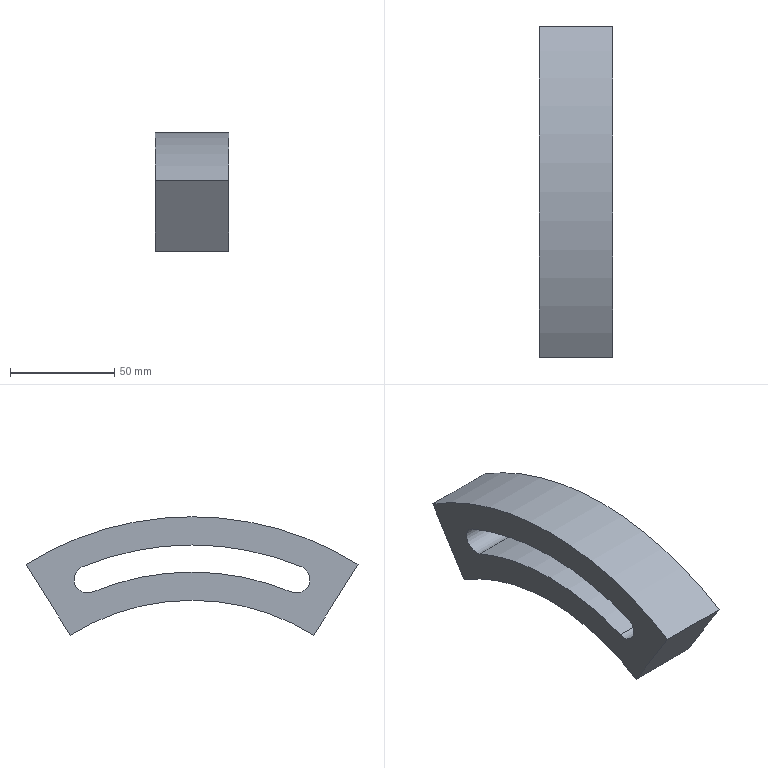Component | NX | COUNTERWEIGHT_BLOCK | 1 solid | 10 faces | box 35 x 158.98 x 56.71 mm | volume 151947 mm3 | cylinder 6 | plane 4 | commonest cylinder face diameters 13 x2 220 x1 300 x1 273 x1 247 x1
STEP:
#1=CARTESIAN_POINT('',(0.,0.,0.));
#2=DIRECTION('',(0.,0.,1.));
#3=DIRECTION('',(1.,0.,0.));
#4=AXIS2_PLACEMENT_3D('',#1,#2,#3);
#5=CARTESIAN_POINT('',(505.625,-79.397,126.65));
#6=VERTEX_POINT('',#5);
#7=CARTESIAN_POINT('',(505.625,-58.2,92.728));
#8=VERTEX_POINT('',#7);
#9=CARTESIAN_POINT('',(505.625,-79.397,126.65));
#10=DIRECTION('',(0.,0.5299,-0.848));
#11=VECTOR('',#10,1.);
#12=LINE('',#9,#11);
#13=CARTESIAN_POINT('',(540.625,-79.397,126.65));
#14=DIRECTION('',(0.,0.848,0.5299));
#15=DIRECTION('',(0.,-0.5299,0.848));
#16=AXIS2_PLACEMENT_3D('',#13,#14,#15);
#17=PLANE('',#16);
#18=CARTESIAN_POINT('',(0.,-35.));
#19=DIRECTION('',(-1.,0.));
#20=VECTOR('',#19,1.);
#21=LINE('',#18,#20);
#22=(GEOMETRIC_REPRESENTATION_CONTEXT(2)PARAMETRIC_REPRESENTATION_CONTEXT()REPRESENTATION_CONTEXT('',''));
#23=DEFINITIONAL_REPRESENTATION('',(#21),#22);
#24=PCURVE('',#17,#23);
#25=CARTESIAN_POINT('',(505.625,0.09065,-0.557));
#26=DIRECTION('',(-1.,0.,0.));
#27=DIRECTION('',(0.,0.,1.));
#28=AXIS2_PLACEMENT_3D('',#25,#26,#27);
#29=PLANE('',#28);
#30=CARTESIAN_POINT('',(127.207,-79.488));
#31=DIRECTION('',(-0.848,0.5299));
#32=VECTOR('',#31,1.);
#33=LINE('',#30,#32);
#34=(GEOMETRIC_REPRESENTATION_CONTEXT(2)PARAMETRIC_REPRESENTATION_CONTEXT()REPRESENTATION_CONTEXT('',''));
#35=DEFINITIONAL_REPRESENTATION('',(#33),#34);
#36=PCURVE('',#29,#35);
#37=SURFACE_CURVE('',#12,(#24,#36),.PCURVE_S1.);
#38=EDGE_CURVE('',#6,#8,#37,.T.);
#39=ORIENTED_EDGE('',*,*,#38,.T.);
#40=CARTESIAN_POINT('',(540.625,-58.2,92.728));
#41=VERTEX_POINT('',#40);
#42=CARTESIAN_POINT('',(540.625,-58.2,92.728));
#43=DIRECTION('',(-1.,0.,0.));
#44=VECTOR('',#43,1.);
#45=LINE('',#42,#44);
#46=CARTESIAN_POINT('',(-40.,0.));
#47=DIRECTION('',(0.,-1.));
#48=VECTOR('',#47,1.);
#49=LINE('',#46,#48);
#50=(GEOMETRIC_REPRESENTATION_CONTEXT(2)PARAMETRIC_REPRESENTATION_CONTEXT()REPRESENTATION_CONTEXT('',''));
#51=DEFINITIONAL_REPRESENTATION('',(#49),#50);
#52=PCURVE('',#17,#51);
#53=CARTESIAN_POINT('',(540.625,0.09065,-0.557));
#54=DIRECTION('',(-1.,0.,0.));
#55=DIRECTION('',(0.,0.,1.));
#56=AXIS2_PLACEMENT_3D('',#53,#54,#55);
#57=CYLINDRICAL_SURFACE('',#56,110.);
#58=CARTESIAN_POINT('',(-0.5585,0.));
#59=DIRECTION('',(0.,1.));
#60=VECTOR('',#59,1.);
#61=LINE('',#58,#60);
#62=(GEOMETRIC_REPRESENTATION_CONTEXT(2)PARAMETRIC_REPRESENTATION_CONTEXT()REPRESENTATION_CONTEXT('',''));
#63=DEFINITIONAL_REPRESENTATION('',(#61),#62);
#64=PCURVE('',#57,#63);
#65=SURFACE_CURVE('',#45,(#52,#64),.PCURVE_S1.);
#66=EDGE_CURVE('',#41,#8,#65,.T.);
#67=ORIENTED_EDGE('',*,*,#66,.F.);
#68=CARTESIAN_POINT('',(540.625,-79.397,126.65));
#69=VERTEX_POINT('',#68);
#70=CARTESIAN_POINT('',(540.625,-79.397,126.65));
#71=DIRECTION('',(0.,0.5299,-0.848));
#72=VECTOR('',#71,1.);
#73=LINE('',#70,#72);
#74=CARTESIAN_POINT('',(0.,0.));
#75=DIRECTION('',(-1.,0.));
#76=VECTOR('',#75,1.);
#77=LINE('',#74,#76);
#78=(GEOMETRIC_REPRESENTATION_CONTEXT(2)PARAMETRIC_REPRESENTATION_CONTEXT()REPRESENTATION_CONTEXT('',''));
#79=DEFINITIONAL_REPRESENTATION('',(#77),#78);
#80=PCURVE('',#17,#79);
#81=CARTESIAN_POINT('',(540.625,0.09065,-0.557));
#82=DIRECTION('',(-1.,0.,0.));
#83=DIRECTION('',(0.,0.,1.));
#84=AXIS2_PLACEMENT_3D('',#81,#82,#83);
#85=PLANE('',#84);
#86=CARTESIAN_POINT('',(127.207,-79.488));
#87=DIRECTION('',(-0.848,0.5299));
#88=VECTOR('',#87,1.);
#89=LINE('',#86,#88);
#90=(GEOMETRIC_REPRESENTATION_CONTEXT(2)PARAMETRIC_REPRESENTATION_CONTEXT()REPRESENTATION_CONTEXT('',''));
#91=DEFINITIONAL_REPRESENTATION('',(#89),#90);
#92=PCURVE('',#85,#91);
#93=SURFACE_CURVE('',#73,(#80,#92),.PCURVE_S1.);
#94=EDGE_CURVE('',#69,#41,#93,.T.);
#95=ORIENTED_EDGE('',*,*,#94,.F.);
#96=CARTESIAN_POINT('',(540.625,-79.397,126.65));
#97=DIRECTION('',(-1.,0.,0.));
#98=VECTOR('',#97,1.);
#99=LINE('',#96,#98);
#100=CARTESIAN_POINT('',(0.,0.));
#101=DIRECTION('',(0.,-1.));
#102=VECTOR('',#101,1.);
#103=LINE('',#100,#102);
#104=(GEOMETRIC_REPRESENTATION_CONTEXT(2)PARAMETRIC_REPRESENTATION_CONTEXT()REPRESENTATION_CONTEXT('',''));
#105=DEFINITIONAL_REPRESENTATION('',(#103),#104);
#106=PCURVE('',#17,#105);
#107=CARTESIAN_POINT('',(540.625,0.09065,-0.557));
#108=DIRECTION('',(-1.,0.,0.));
#109=DIRECTION('',(0.,0.,1.));
#110=AXIS2_PLACEMENT_3D('',#107,#108,#109);
#111=CYLINDRICAL_SURFACE('',#110,150.);
#112=CARTESIAN_POINT('',(-0.5585,0.));
#113=DIRECTION('',(0.,1.));
#114=VECTOR('',#113,1.);
#115=LINE('',#112,#114);
#116=(GEOMETRIC_REPRESENTATION_CONTEXT(2)PARAMETRIC_REPRESENTATION_CONTEXT()REPRESENTATION_CONTEXT('',''));
#117=DEFINITIONAL_REPRESENTATION('',(#115),#116);
#118=PCURVE('',#111,#117);
#119=SURFACE_CURVE('',#99,(#106,#118),.PCURVE_S1.);
#120=EDGE_CURVE('',#69,#6,#119,.T.);
#121=ORIENTED_EDGE('',*,*,#120,.T.);
#122=EDGE_LOOP('',(#39,#67,#95,#121));
#123=FACE_BOUND('',#122,.T.);
#124=ADVANCED_FACE('',(#123),#17,.F.);
#125=ORIENTED_EDGE('',*,*,#66,.F.);
#126=CARTESIAN_POINT('',(540.625,58.382,92.728));
#127=VERTEX_POINT('',#126);
#128=CARTESIAN_POINT('',(540.625,0.09065,-0.557));
#129=DIRECTION('',(-1.,0.,0.));
#130=DIRECTION('',(0.,1.,0.));
#131=AXIS2_PLACEMENT_3D('',#128,#129,#130);
#132=CIRCLE('',#131,110.);
#133=CARTESIAN_POINT('',(-4.712,0.));
#134=DIRECTION('',(1.,0.));
#135=VECTOR('',#134,1.);
#136=LINE('',#133,#135);
#137=(GEOMETRIC_REPRESENTATION_CONTEXT(2)PARAMETRIC_REPRESENTATION_CONTEXT()REPRESENTATION_CONTEXT('',''));
#138=DEFINITIONAL_REPRESENTATION('',(#136),#137);
#139=PCURVE('',#57,#138);
#140=CARTESIAN_POINT('',(0.,0.));
#141=DIRECTION('',(0.,1.));
#142=AXIS2_PLACEMENT_2D('',#140,#141);
#143=CIRCLE('',#142,110.);
#144=(GEOMETRIC_REPRESENTATION_CONTEXT(2)PARAMETRIC_REPRESENTATION_CONTEXT()REPRESENTATION_CONTEXT('',''));
#145=DEFINITIONAL_REPRESENTATION('',(#143),#144);
#146=PCURVE('',#85,#145);
#147=SURFACE_CURVE('',#132,(#139,#146),.PCURVE_S1.);
#148=EDGE_CURVE('',#41,#127,#147,.T.);
#149=ORIENTED_EDGE('',*,*,#148,.T.);
#150=CARTESIAN_POINT('',(505.625,58.382,92.728));
#151=VERTEX_POINT('',#150);
#152=CARTESIAN_POINT('',(540.625,58.382,92.728));
#153=DIRECTION('',(-1.,0.,0.));
#154=VECTOR('',#153,1.);
#155=LINE('',#152,#154);
#156=CARTESIAN_POINT('',(0.5585,0.));
#157=DIRECTION('',(0.,1.));
#158=VECTOR('',#157,1.);
#159=LINE('',#156,#158);
#160=(GEOMETRIC_REPRESENTATION_CONTEXT(2)PARAMETRIC_REPRESENTATION_CONTEXT()REPRESENTATION_CONTEXT('',''));
#161=DEFINITIONAL_REPRESENTATION('',(#159),#160);
#162=PCURVE('',#57,#161);
#163=CARTESIAN_POINT('',(540.625,58.382,92.728));
#164=DIRECTION('',(0.,-0.848,0.5299));
#165=DIRECTION('',(0.,-0.5299,-0.848));
#166=AXIS2_PLACEMENT_3D('',#163,#164,#165);
#167=PLANE('',#166);
#168=CARTESIAN_POINT('',(0.,0.));
#169=DIRECTION('',(0.,-1.));
#170=VECTOR('',#169,1.);
#171=LINE('',#168,#170);
#172=(GEOMETRIC_REPRESENTATION_CONTEXT(2)PARAMETRIC_REPRESENTATION_CONTEXT()REPRESENTATION_CONTEXT('',''));
#173=DEFINITIONAL_REPRESENTATION('',(#171),#172);
#174=PCURVE('',#167,#173);
#175=SURFACE_CURVE('',#155,(#162,#174),.PCURVE_S1.);
#176=EDGE_CURVE('',#127,#151,#175,.T.);
#177=ORIENTED_EDGE('',*,*,#176,.T.);
#178=CARTESIAN_POINT('',(505.625,0.09065,-0.557));
#179=DIRECTION('',(-1.,0.,0.));
#180=DIRECTION('',(0.,1.,0.));
#181=AXIS2_PLACEMENT_3D('',#178,#179,#180);
#182=CIRCLE('',#181,110.);
#183=CARTESIAN_POINT('',(-4.712,35.));
#184=DIRECTION('',(1.,0.));
#185=VECTOR('',#184,1.);
#186=LINE('',#183,#185);
#187=(GEOMETRIC_REPRESENTATION_CONTEXT(2)PARAMETRIC_REPRESENTATION_CONTEXT()REPRESENTATION_CONTEXT('',''));
#188=DEFINITIONAL_REPRESENTATION('',(#186),#187);
#189=PCURVE('',#57,#188);
#190=CARTESIAN_POINT('',(0.,0.));
#191=DIRECTION('',(0.,1.));
#192=AXIS2_PLACEMENT_2D('',#190,#191);
#193=CIRCLE('',#192,110.);
#194=(GEOMETRIC_REPRESENTATION_CONTEXT(2)PARAMETRIC_REPRESENTATION_CONTEXT()REPRESENTATION_CONTEXT('',''));
#195=DEFINITIONAL_REPRESENTATION('',(#193),#194);
#196=PCURVE('',#29,#195);
#197=SURFACE_CURVE('',#182,(#189,#196),.PCURVE_S1.);
#198=EDGE_CURVE('',#8,#151,#197,.T.);
#199=ORIENTED_EDGE('',*,*,#198,.F.);
#200=EDGE_LOOP('',(#125,#149,#177,#199));
#201=FACE_BOUND('',#200,.F.);
#202=ADVANCED_FACE('',(#201),#57,.F.);
#203=CARTESIAN_POINT('',(505.625,79.579,126.65));
#204=VERTEX_POINT('',#203);
#205=CARTESIAN_POINT('',(505.625,58.382,92.728));
#206=DIRECTION('',(0.,0.5299,0.848));
#207=VECTOR('',#206,1.);
#208=LINE('',#205,#207);
#209=CARTESIAN_POINT('',(0.,-35.));
#210=DIRECTION('',(-1.,0.));
#211=VECTOR('',#210,1.);
#212=LINE('',#209,#211);
#213=(GEOMETRIC_REPRESENTATION_CONTEXT(2)PARAMETRIC_REPRESENTATION_CONTEXT()REPRESENTATION_CONTEXT('',''));
#214=DEFINITIONAL_REPRESENTATION('',(#212),#213);
#215=PCURVE('',#167,#214);
#216=CARTESIAN_POINT('',(93.285,58.291));
#217=DIRECTION('',(0.848,0.5299));
#218=VECTOR('',#217,1.);
#219=LINE('',#216,#218);
#220=(GEOMETRIC_REPRESENTATION_CONTEXT(2)PARAMETRIC_REPRESENTATION_CONTEXT()REPRESENTATION_CONTEXT('',''));
#221=DEFINITIONAL_REPRESENTATION('',(#219),#220);
#222=PCURVE('',#29,#221);
#223=SURFACE_CURVE('',#208,(#215,#222),.PCURVE_S1.);
#224=EDGE_CURVE('',#151,#204,#223,.T.);
#225=ORIENTED_EDGE('',*,*,#224,.T.);
#226=CARTESIAN_POINT('',(540.625,79.579,126.65));
#227=VERTEX_POINT('',#226);
#228=CARTESIAN_POINT('',(540.625,79.579,126.65));
#229=DIRECTION('',(-1.,0.,0.));
#230=VECTOR('',#229,1.);
#231=LINE('',#228,#230);
#232=CARTESIAN_POINT('',(-40.,0.));
#233=DIRECTION('',(0.,-1.));
#234=VECTOR('',#233,1.);
#235=LINE('',#232,#234);
#236=(GEOMETRIC_REPRESENTATION_CONTEXT(2)PARAMETRIC_REPRESENTATION_CONTEXT()REPRESENTATION_CONTEXT('',''));
#237=DEFINITIONAL_REPRESENTATION('',(#235),#236);
#238=PCURVE('',#167,#237);
#239=CARTESIAN_POINT('',(0.5585,0.));
#240=DIRECTION('',(0.,1.));
#241=VECTOR('',#240,1.);
#242=LINE('',#239,#241);
#243=(GEOMETRIC_REPRESENTATION_CONTEXT(2)PARAMETRIC_REPRESENTATION_CONTEXT()REPRESENTATION_CONTEXT('',''));
#244=DEFINITIONAL_REPRESENTATION('',(#242),#243);
#245=PCURVE('',#111,#244);
#246=SURFACE_CURVE('',#231,(#238,#245),.PCURVE_S1.);
#247=EDGE_CURVE('',#227,#204,#246,.T.);
#248=ORIENTED_EDGE('',*,*,#247,.F.);
#249=CARTESIAN_POINT('',(540.625,58.382,92.728));
#250=DIRECTION('',(0.,0.5299,0.848));
#251=VECTOR('',#250,1.);
#252=LINE('',#249,#251);
#253=CARTESIAN_POINT('',(0.,0.));
#254=DIRECTION('',(-1.,0.));
#255=VECTOR('',#254,1.);
#256=LINE('',#253,#255);
#257=(GEOMETRIC_REPRESENTATION_CONTEXT(2)PARAMETRIC_REPRESENTATION_CONTEXT()REPRESENTATION_CONTEXT('',''));
#258=DEFINITIONAL_REPRESENTATION('',(#256),#257);
#259=PCURVE('',#167,#258);
#260=CARTESIAN_POINT('',(93.285,58.291));
#261=DIRECTION('',(0.848,0.5299));
#262=VECTOR('',#261,1.);
#263=LINE('',#260,#262);
#264=(GEOMETRIC_REPRESENTATION_CONTEXT(2)PARAMETRIC_REPRESENTATION_CONTEXT()REPRESENTATION_CONTEXT('',''));
#265=DEFINITIONAL_REPRESENTATION('',(#263),#264);
#266=PCURVE('',#85,#265);
#267=SURFACE_CURVE('',#252,(#259,#266),.PCURVE_S1.);
#268=EDGE_CURVE('',#127,#227,#267,.T.);
#269=ORIENTED_EDGE('',*,*,#268,.F.);
#270=ORIENTED_EDGE('',*,*,#176,.T.);
#271=EDGE_LOOP('',(#225,#248,#269,#270));
#272=FACE_BOUND('',#271,.T.);
#273=ADVANCED_FACE('',(#272),#167,.F.);
#274=CARTESIAN_POINT('',(505.625,0.09065,-0.557));
#275=DIRECTION('',(1.,0.,0.));
#276=DIRECTION('',(0.,1.,-0.));
#277=AXIS2_PLACEMENT_3D('',#274,#275,#276);
#278=CIRCLE('',#277,150.);
#279=CARTESIAN_POINT('',(1.571,35.));
#280=DIRECTION('',(-1.,0.));
#281=VECTOR('',#280,1.);
#282=LINE('',#279,#281);
#283=(GEOMETRIC_REPRESENTATION_CONTEXT(2)PARAMETRIC_REPRESENTATION_CONTEXT()REPRESENTATION_CONTEXT('',''));
#284=DEFINITIONAL_REPRESENTATION('',(#282),#283);
#285=PCURVE('',#111,#284);
#286=CARTESIAN_POINT('',(-0.,150.));
#287=CARTESIAN_POINT('',(259.808,150.));
#288=CARTESIAN_POINT('',(129.904,-75.));
#289=CARTESIAN_POINT('',(0.,-300.));
#290=CARTESIAN_POINT('',(-129.904,-75.));
#291=CARTESIAN_POINT('',(-259.808,150.));
#292=CARTESIAN_POINT('',(-0.,150.));
#293=(BOUNDED_CURVE()B_SPLINE_CURVE(2,(#286,#287,#288,#289,#290,#291,#292),.UNSPECIFIED.,.T.,.F.)B_SPLINE_CURVE_WITH_KNOTS((1,2,2,2,2,1),(-2.094,0.,2.094,4.189,6.283,8.378),.UNSPECIFIED.)CURVE()GEOMETRIC_REPRESENTATION_ITEM()RATIONAL_B_SPLINE_CURVE((1.,0.5,1.,0.5,1.,0.5,1.))REPRESENTATION_ITEM(''));
#294=(GEOMETRIC_REPRESENTATION_CONTEXT(2)PARAMETRIC_REPRESENTATION_CONTEXT()REPRESENTATION_CONTEXT('',''));
#295=DEFINITIONAL_REPRESENTATION('',(#293),#294);
#296=PCURVE('',#29,#295);
#297=SURFACE_CURVE('',#278,(#285,#296),.PCURVE_S1.);
#298=EDGE_CURVE('',#204,#6,#297,.T.);
#299=ORIENTED_EDGE('',*,*,#298,.T.);
#300=ORIENTED_EDGE('',*,*,#120,.F.);
#301=CARTESIAN_POINT('',(540.625,0.09065,-0.557));
#302=DIRECTION('',(1.,0.,0.));
#303=DIRECTION('',(0.,1.,-0.));
#304=AXIS2_PLACEMENT_3D('',#301,#302,#303);
#305=CIRCLE('',#304,150.);
#306=CARTESIAN_POINT('',(1.571,0.));
#307=DIRECTION('',(-1.,0.));
#308=VECTOR('',#307,1.);
#309=LINE('',#306,#308);
#310=(GEOMETRIC_REPRESENTATION_CONTEXT(2)PARAMETRIC_REPRESENTATION_CONTEXT()REPRESENTATION_CONTEXT('',''));
#311=DEFINITIONAL_REPRESENTATION('',(#309),#310);
#312=PCURVE('',#111,#311);
#313=CARTESIAN_POINT('',(-0.,150.));
#314=CARTESIAN_POINT('',(259.808,150.));
#315=CARTESIAN_POINT('',(129.904,-75.));
#316=CARTESIAN_POINT('',(0.,-300.));
#317=CARTESIAN_POINT('',(-129.904,-75.));
#318=CARTESIAN_POINT('',(-259.808,150.));
#319=CARTESIAN_POINT('',(-0.,150.));
#320=(BOUNDED_CURVE()B_SPLINE_CURVE(2,(#313,#314,#315,#316,#317,#318,#319),.UNSPECIFIED.,.T.,.F.)B_SPLINE_CURVE_WITH_KNOTS((1,2,2,2,2,1),(-2.094,0.,2.094,4.189,6.283,8.378),.UNSPECIFIED.)CURVE()GEOMETRIC_REPRESENTATION_ITEM()RATIONAL_B_SPLINE_CURVE((1.,0.5,1.,0.5,1.,0.5,1.))REPRESENTATION_ITEM(''));
#321=(GEOMETRIC_REPRESENTATION_CONTEXT(2)PARAMETRIC_REPRESENTATION_CONTEXT()REPRESENTATION_CONTEXT('',''));
#322=DEFINITIONAL_REPRESENTATION('',(#320),#321);
#323=PCURVE('',#85,#322);
#324=SURFACE_CURVE('',#305,(#312,#323),.PCURVE_S1.);
#325=EDGE_CURVE('',#227,#69,#324,.T.);
#326=ORIENTED_EDGE('',*,*,#325,.F.);
#327=ORIENTED_EDGE('',*,*,#247,.T.);
#328=EDGE_LOOP('',(#299,#300,#326,#327));
#329=FACE_BOUND('',#328,.T.);
#330=ADVANCED_FACE('',(#329),#111,.T.);
#331=CARTESIAN_POINT('',(540.625,-52.409,125.443));
#332=VERTEX_POINT('',#331);
#333=CARTESIAN_POINT('',(540.625,52.591,125.443));
#334=VERTEX_POINT('',#333);
#335=CARTESIAN_POINT('',(540.625,0.09065,-0.557));
#336=DIRECTION('',(-1.,0.,0.));
#337=DIRECTION('',(0.,1.,0.));
#338=AXIS2_PLACEMENT_3D('',#335,#336,#337);
#339=CIRCLE('',#338,136.5);
#340=CARTESIAN_POINT('',(0.,0.));
#341=DIRECTION('',(0.,1.));
#342=AXIS2_PLACEMENT_2D('',#340,#341);
#343=CIRCLE('',#342,136.5);
#344=(GEOMETRIC_REPRESENTATION_CONTEXT(2)PARAMETRIC_REPRESENTATION_CONTEXT()REPRESENTATION_CONTEXT('',''));
#345=DEFINITIONAL_REPRESENTATION('',(#343),#344);
#346=PCURVE('',#85,#345);
#347=CARTESIAN_POINT('',(500.625,0.09065,-0.557));
#348=DIRECTION('',(1.,0.,0.));
#349=DIRECTION('',(0.,0.,-1.));
#350=AXIS2_PLACEMENT_3D('',#347,#348,#349);
#351=CYLINDRICAL_SURFACE('',#350,136.5);
#352=CARTESIAN_POINT('',(7.854,40.));
#353=DIRECTION('',(-1.,0.));
#354=VECTOR('',#353,1.);
#355=LINE('',#352,#354);
#356=(GEOMETRIC_REPRESENTATION_CONTEXT(2)PARAMETRIC_REPRESENTATION_CONTEXT()REPRESENTATION_CONTEXT('',''));
#357=DEFINITIONAL_REPRESENTATION('',(#355),#356);
#358=PCURVE('',#351,#357);
#359=SURFACE_CURVE('',#339,(#346,#358),.PCURVE_S1.);
#360=EDGE_CURVE('',#332,#334,#359,.T.);
#361=ORIENTED_EDGE('',*,*,#360,.T.);
#362=CARTESIAN_POINT('',(540.625,47.591,113.443));
#363=VERTEX_POINT('',#362);
#364=CARTESIAN_POINT('',(540.625,50.091,119.443));
#365=DIRECTION('',(-1.,0.,0.));
#366=DIRECTION('',(0.,1.,0.));
#367=AXIS2_PLACEMENT_3D('',#364,#365,#366);
#368=CIRCLE('',#367,6.5);
#369=CARTESIAN_POINT('',(120.,50.));
#370=DIRECTION('',(0.,1.));
#371=AXIS2_PLACEMENT_2D('',#369,#370);
#372=CIRCLE('',#371,6.5);
#373=(GEOMETRIC_REPRESENTATION_CONTEXT(2)PARAMETRIC_REPRESENTATION_CONTEXT()REPRESENTATION_CONTEXT('',''));
#374=DEFINITIONAL_REPRESENTATION('',(#372),#373);
#375=PCURVE('',#85,#374);
#376=CARTESIAN_POINT('',(500.625,50.091,119.443));
#377=DIRECTION('',(1.,0.,0.));
#378=DIRECTION('',(0.,0.,-1.));
#379=AXIS2_PLACEMENT_3D('',#376,#377,#378);
#380=CYLINDRICAL_SURFACE('',#379,6.5);
#381=CARTESIAN_POINT('',(7.854,40.));
#382=DIRECTION('',(-1.,0.));
#383=VECTOR('',#382,1.);
#384=LINE('',#381,#383);
#385=(GEOMETRIC_REPRESENTATION_CONTEXT(2)PARAMETRIC_REPRESENTATION_CONTEXT()REPRESENTATION_CONTEXT('',''));
#386=DEFINITIONAL_REPRESENTATION('',(#384),#385);
#387=PCURVE('',#380,#386);
#388=SURFACE_CURVE('',#368,(#375,#387),.PCURVE_S1.);
#389=EDGE_CURVE('',#334,#363,#388,.T.);
#390=ORIENTED_EDGE('',*,*,#389,.T.);
#391=CARTESIAN_POINT('',(540.625,-47.409,113.443));
#392=VERTEX_POINT('',#391);
#393=CARTESIAN_POINT('',(540.625,0.09065,-0.557));
#394=DIRECTION('',(1.,0.,0.));
#395=DIRECTION('',(0.,1.,-0.));
#396=AXIS2_PLACEMENT_3D('',#393,#394,#395);
#397=CIRCLE('',#396,123.5);
#398=CARTESIAN_POINT('',(-0.,123.5));
#399=CARTESIAN_POINT('',(213.908,123.5));
#400=CARTESIAN_POINT('',(106.954,-61.75));
#401=CARTESIAN_POINT('',(0.,-247.));
#402=CARTESIAN_POINT('',(-106.954,-61.75));
#403=CARTESIAN_POINT('',(-213.908,123.5));
#404=CARTESIAN_POINT('',(-0.,123.5));
#405=(BOUNDED_CURVE()B_SPLINE_CURVE(2,(#398,#399,#400,#401,#402,#403,#404),.UNSPECIFIED.,.T.,.F.)B_SPLINE_CURVE_WITH_KNOTS((1,2,2,2,2,1),(-2.094,0.,2.094,4.189,6.283,8.378),.UNSPECIFIED.)CURVE()GEOMETRIC_REPRESENTATION_ITEM()RATIONAL_B_SPLINE_CURVE((1.,0.5,1.,0.5,1.,0.5,1.))REPRESENTATION_ITEM(''));
#406=(GEOMETRIC_REPRESENTATION_CONTEXT(2)PARAMETRIC_REPRESENTATION_CONTEXT()REPRESENTATION_CONTEXT('',''));
#407=DEFINITIONAL_REPRESENTATION('',(#405),#406);
#408=PCURVE('',#85,#407);
#409=CARTESIAN_POINT('',(500.625,0.09065,-0.557));
#410=DIRECTION('',(1.,0.,0.));
#411=DIRECTION('',(0.,0.,-1.));
#412=AXIS2_PLACEMENT_3D('',#409,#410,#411);
#413=CYLINDRICAL_SURFACE('',#412,123.5);
#414=CARTESIAN_POINT('',(1.571,40.));
#415=DIRECTION('',(1.,0.));
#416=VECTOR('',#415,1.);
#417=LINE('',#414,#416);
#418=(GEOMETRIC_REPRESENTATION_CONTEXT(2)PARAMETRIC_REPRESENTATION_CONTEXT()REPRESENTATION_CONTEXT('',''));
#419=DEFINITIONAL_REPRESENTATION('',(#417),#418);
#420=PCURVE('',#413,#419);
#421=SURFACE_CURVE('',#397,(#408,#420),.PCURVE_S1.);
#422=EDGE_CURVE('',#363,#392,#421,.T.);
#423=ORIENTED_EDGE('',*,*,#422,.T.);
#424=CARTESIAN_POINT('',(540.625,-49.909,119.443));
#425=DIRECTION('',(-1.,0.,0.));
#426=DIRECTION('',(0.,1.,0.));
#427=AXIS2_PLACEMENT_3D('',#424,#425,#426);
#428=CIRCLE('',#427,6.5);
#429=CARTESIAN_POINT('',(120.,-50.));
#430=DIRECTION('',(0.,1.));
#431=AXIS2_PLACEMENT_2D('',#429,#430);
#432=CIRCLE('',#431,6.5);
#433=(GEOMETRIC_REPRESENTATION_CONTEXT(2)PARAMETRIC_REPRESENTATION_CONTEXT()REPRESENTATION_CONTEXT('',''));
#434=DEFINITIONAL_REPRESENTATION('',(#432),#433);
#435=PCURVE('',#85,#434);
#436=CARTESIAN_POINT('',(500.625,-49.909,119.443));
#437=DIRECTION('',(1.,0.,0.));
#438=DIRECTION('',(0.,0.,-1.));
#439=AXIS2_PLACEMENT_3D('',#436,#437,#438);
#440=CYLINDRICAL_SURFACE('',#439,6.5);
#441=CARTESIAN_POINT('',(7.854,40.));
#442=DIRECTION('',(-1.,0.));
#443=VECTOR('',#442,1.);
#444=LINE('',#441,#443);
#445=(GEOMETRIC_REPRESENTATION_CONTEXT(2)PARAMETRIC_REPRESENTATION_CONTEXT()REPRESENTATION_CONTEXT('',''));
#446=DEFINITIONAL_REPRESENTATION('',(#444),#445);
#447=PCURVE('',#440,#446);
#448=SURFACE_CURVE('',#428,(#435,#447),.PCURVE_S1.);
#449=EDGE_CURVE('',#392,#332,#448,.T.);
#450=ORIENTED_EDGE('',*,*,#449,.T.);
#451=EDGE_LOOP('',(#361,#390,#423,#450));
#452=FACE_BOUND('',#451,.T.);
#453=ORIENTED_EDGE('',*,*,#94,.T.);
#454=ORIENTED_EDGE('',*,*,#148,.T.);
#455=ORIENTED_EDGE('',*,*,#268,.T.);
#456=ORIENTED_EDGE('',*,*,#325,.T.);
#457=EDGE_LOOP('',(#453,#454,#455,#456));
#458=FACE_BOUND('',#457,.T.);
#459=ADVANCED_FACE('',(#452,#458),#85,.F.);
#460=CARTESIAN_POINT('',(505.625,47.591,113.443));
#461=VERTEX_POINT('',#460);
#462=CARTESIAN_POINT('',(505.625,52.591,125.443));
#463=VERTEX_POINT('',#462);
#464=CARTESIAN_POINT('',(505.625,50.091,119.443));
#465=DIRECTION('',(1.,0.,0.));
#466=DIRECTION('',(0.,0.,1.));
#467=AXIS2_PLACEMENT_3D('',#464,#465,#466);
#468=CIRCLE('',#467,6.5);
#469=CARTESIAN_POINT('',(126.5,50.));
#470=CARTESIAN_POINT('',(126.5,38.742));
#471=CARTESIAN_POINT('',(116.75,44.371));
#472=CARTESIAN_POINT('',(107.,50.));
#473=CARTESIAN_POINT('',(116.75,55.629));
#474=CARTESIAN_POINT('',(126.5,61.258));
#475=CARTESIAN_POINT('',(126.5,50.));
#476=(BOUNDED_CURVE()B_SPLINE_CURVE(2,(#469,#470,#471,#472,#473,#474,#475),.UNSPECIFIED.,.T.,.F.)B_SPLINE_CURVE_WITH_KNOTS((1,2,2,2,2,1),(-2.094,0.,2.094,4.189,6.283,8.378),.UNSPECIFIED.)CURVE()GEOMETRIC_REPRESENTATION_ITEM()RATIONAL_B_SPLINE_CURVE((1.,0.5,1.,0.5,1.,0.5,1.))REPRESENTATION_ITEM(''));
#477=(GEOMETRIC_REPRESENTATION_CONTEXT(2)PARAMETRIC_REPRESENTATION_CONTEXT()REPRESENTATION_CONTEXT('',''));
#478=DEFINITIONAL_REPRESENTATION('',(#476),#477);
#479=PCURVE('',#29,#478);
#480=CARTESIAN_POINT('',(-3.142,5.));
#481=DIRECTION('',(1.,0.));
#482=VECTOR('',#481,1.);
#483=LINE('',#480,#482);
#484=(GEOMETRIC_REPRESENTATION_CONTEXT(2)PARAMETRIC_REPRESENTATION_CONTEXT()REPRESENTATION_CONTEXT('',''));
#485=DEFINITIONAL_REPRESENTATION('',(#483),#484);
#486=PCURVE('',#380,#485);
#487=SURFACE_CURVE('',#468,(#479,#486),.PCURVE_S1.);
#488=EDGE_CURVE('',#461,#463,#487,.T.);
#489=ORIENTED_EDGE('',*,*,#488,.T.);
#490=CARTESIAN_POINT('',(505.625,-52.409,125.443));
#491=VERTEX_POINT('',#490);
#492=CARTESIAN_POINT('',(505.625,0.09065,-0.557));
#493=DIRECTION('',(1.,0.,0.));
#494=DIRECTION('',(0.,0.,1.));
#495=AXIS2_PLACEMENT_3D('',#492,#493,#494);
#496=CIRCLE('',#495,136.5);
#497=CARTESIAN_POINT('',(136.5,0.));
#498=CARTESIAN_POINT('',(136.5,-236.425));
#499=CARTESIAN_POINT('',(-68.25,-118.212));
#500=CARTESIAN_POINT('',(-273.,-0.));
#501=CARTESIAN_POINT('',(-68.25,118.212));
#502=CARTESIAN_POINT('',(136.5,236.425));
#503=CARTESIAN_POINT('',(136.5,0.));
#504=(BOUNDED_CURVE()B_SPLINE_CURVE(2,(#497,#498,#499,#500,#501,#502,#503),.UNSPECIFIED.,.T.,.F.)B_SPLINE_CURVE_WITH_KNOTS((1,2,2,2,2,1),(-2.094,0.,2.094,4.189,6.283,8.378),.UNSPECIFIED.)CURVE()GEOMETRIC_REPRESENTATION_ITEM()RATIONAL_B_SPLINE_CURVE((1.,0.5,1.,0.5,1.,0.5,1.))REPRESENTATION_ITEM(''));
#505=(GEOMETRIC_REPRESENTATION_CONTEXT(2)PARAMETRIC_REPRESENTATION_CONTEXT()REPRESENTATION_CONTEXT('',''));
#506=DEFINITIONAL_REPRESENTATION('',(#504),#505);
#507=PCURVE('',#29,#506);
#508=CARTESIAN_POINT('',(-3.142,5.));
#509=DIRECTION('',(1.,0.));
#510=VECTOR('',#509,1.);
#511=LINE('',#508,#510);
#512=(GEOMETRIC_REPRESENTATION_CONTEXT(2)PARAMETRIC_REPRESENTATION_CONTEXT()REPRESENTATION_CONTEXT('',''));
#513=DEFINITIONAL_REPRESENTATION('',(#511),#512);
#514=PCURVE('',#351,#513);
#515=SURFACE_CURVE('',#496,(#507,#514),.PCURVE_S1.);
#516=EDGE_CURVE('',#463,#491,#515,.T.);
#517=ORIENTED_EDGE('',*,*,#516,.T.);
#518=CARTESIAN_POINT('',(505.625,-47.409,113.443));
#519=VERTEX_POINT('',#518);
#520=CARTESIAN_POINT('',(505.625,-49.909,119.443));
#521=DIRECTION('',(1.,0.,0.));
#522=DIRECTION('',(0.,0.,1.));
#523=AXIS2_PLACEMENT_3D('',#520,#521,#522);
#524=CIRCLE('',#523,6.5);
#525=CARTESIAN_POINT('',(126.5,-50.));
#526=CARTESIAN_POINT('',(126.5,-61.258));
#527=CARTESIAN_POINT('',(116.75,-55.629));
#528=CARTESIAN_POINT('',(107.,-50.));
#529=CARTESIAN_POINT('',(116.75,-44.371));
#530=CARTESIAN_POINT('',(126.5,-38.742));
#531=CARTESIAN_POINT('',(126.5,-50.));
#532=(BOUNDED_CURVE()B_SPLINE_CURVE(2,(#525,#526,#527,#528,#529,#530,#531),.UNSPECIFIED.,.T.,.F.)B_SPLINE_CURVE_WITH_KNOTS((1,2,2,2,2,1),(-2.094,0.,2.094,4.189,6.283,8.378),.UNSPECIFIED.)CURVE()GEOMETRIC_REPRESENTATION_ITEM()RATIONAL_B_SPLINE_CURVE((1.,0.5,1.,0.5,1.,0.5,1.))REPRESENTATION_ITEM(''));
#533=(GEOMETRIC_REPRESENTATION_CONTEXT(2)PARAMETRIC_REPRESENTATION_CONTEXT()REPRESENTATION_CONTEXT('',''));
#534=DEFINITIONAL_REPRESENTATION('',(#532),#533);
#535=PCURVE('',#29,#534);
#536=CARTESIAN_POINT('',(3.142,5.));
#537=DIRECTION('',(1.,0.));
#538=VECTOR('',#537,1.);
#539=LINE('',#536,#538);
#540=(GEOMETRIC_REPRESENTATION_CONTEXT(2)PARAMETRIC_REPRESENTATION_CONTEXT()REPRESENTATION_CONTEXT('',''));
#541=DEFINITIONAL_REPRESENTATION('',(#539),#540);
#542=PCURVE('',#440,#541);
#543=SURFACE_CURVE('',#524,(#535,#542),.PCURVE_S1.);
#544=EDGE_CURVE('',#491,#519,#543,.T.);
#545=ORIENTED_EDGE('',*,*,#544,.T.);
#546=CARTESIAN_POINT('',(505.625,0.09065,-0.557));
#547=DIRECTION('',(-1.,0.,0.));
#548=DIRECTION('',(0.,0.,1.));
#549=AXIS2_PLACEMENT_3D('',#546,#547,#548);
#550=CIRCLE('',#549,123.5);
#551=CARTESIAN_POINT('',(0.,0.));
#552=DIRECTION('',(1.,0.));
#553=AXIS2_PLACEMENT_2D('',#551,#552);
#554=CIRCLE('',#553,123.5);
#555=(GEOMETRIC_REPRESENTATION_CONTEXT(2)PARAMETRIC_REPRESENTATION_CONTEXT()REPRESENTATION_CONTEXT('',''));
#556=DEFINITIONAL_REPRESENTATION('',(#554),#555);
#557=PCURVE('',#29,#556);
#558=CARTESIAN_POINT('',(9.425,5.));
#559=DIRECTION('',(-1.,0.));
#560=VECTOR('',#559,1.);
#561=LINE('',#558,#560);
#562=(GEOMETRIC_REPRESENTATION_CONTEXT(2)PARAMETRIC_REPRESENTATION_CONTEXT()REPRESENTATION_CONTEXT('',''));
#563=DEFINITIONAL_REPRESENTATION('',(#561),#562);
#564=PCURVE('',#413,#563);
#565=SURFACE_CURVE('',#550,(#557,#564),.PCURVE_S1.);
#566=EDGE_CURVE('',#519,#461,#565,.T.);
#567=ORIENTED_EDGE('',*,*,#566,.T.);
#568=EDGE_LOOP('',(#489,#517,#545,#567));
#569=FACE_BOUND('',#568,.T.);
#570=ORIENTED_EDGE('',*,*,#38,.F.);
#571=ORIENTED_EDGE('',*,*,#298,.F.);
#572=ORIENTED_EDGE('',*,*,#224,.F.);
#573=ORIENTED_EDGE('',*,*,#198,.F.);
#574=EDGE_LOOP('',(#570,#571,#572,#573));
#575=FACE_BOUND('',#574,.T.);
#576=ADVANCED_FACE('',(#569,#575),#29,.T.);
#577=ORIENTED_EDGE('',*,*,#516,.T.);
#578=CARTESIAN_POINT('',(500.625,-52.409,125.443));
#579=DIRECTION('',(-1.,0.,0.));
#580=VECTOR('',#579,1.);
#581=LINE('',#578,#580);
#582=CARTESIAN_POINT('',(3.536,0.));
#583=DIRECTION('',(0.,-1.));
#584=VECTOR('',#583,1.);
#585=LINE('',#582,#584);
#586=(GEOMETRIC_REPRESENTATION_CONTEXT(2)PARAMETRIC_REPRESENTATION_CONTEXT()REPRESENTATION_CONTEXT('',''));
#587=DEFINITIONAL_REPRESENTATION('',(#585),#586);
#588=PCURVE('',#351,#587);
#589=CARTESIAN_POINT('',(3.536,0.));
#590=DIRECTION('',(0.,-1.));
#591=VECTOR('',#590,1.);
#592=LINE('',#589,#591);
#593=(GEOMETRIC_REPRESENTATION_CONTEXT(2)PARAMETRIC_REPRESENTATION_CONTEXT()REPRESENTATION_CONTEXT('',''));
#594=DEFINITIONAL_REPRESENTATION('',(#592),#593);
#595=PCURVE('',#440,#594);
#596=SURFACE_CURVE('',#581,(#588,#595),.PCURVE_S1.);
#597=EDGE_CURVE('',#332,#491,#596,.T.);
#598=ORIENTED_EDGE('',*,*,#597,.F.);
#599=ORIENTED_EDGE('',*,*,#360,.T.);
#600=CARTESIAN_POINT('',(500.625,52.591,125.443));
#601=DIRECTION('',(-1.,0.,0.));
#602=VECTOR('',#601,1.);
#603=LINE('',#600,#602);
#604=CARTESIAN_POINT('',(2.747,0.));
#605=DIRECTION('',(0.,-1.));
#606=VECTOR('',#605,1.);
#607=LINE('',#604,#606);
#608=(GEOMETRIC_REPRESENTATION_CONTEXT(2)PARAMETRIC_REPRESENTATION_CONTEXT()REPRESENTATION_CONTEXT('',''));
#609=DEFINITIONAL_REPRESENTATION('',(#607),#608);
#610=PCURVE('',#351,#609);
#611=CARTESIAN_POINT('',(2.747,0.));
#612=DIRECTION('',(0.,-1.));
#613=VECTOR('',#612,1.);
#614=LINE('',#611,#613);
#615=(GEOMETRIC_REPRESENTATION_CONTEXT(2)PARAMETRIC_REPRESENTATION_CONTEXT()REPRESENTATION_CONTEXT('',''));
#616=DEFINITIONAL_REPRESENTATION('',(#614),#615);
#617=PCURVE('',#380,#616);
#618=SURFACE_CURVE('',#603,(#610,#617),.PCURVE_S1.);
#619=EDGE_CURVE('',#334,#463,#618,.T.);
#620=ORIENTED_EDGE('',*,*,#619,.T.);
#621=EDGE_LOOP('',(#577,#598,#599,#620));
#622=FACE_BOUND('',#621,.F.);
#623=ADVANCED_FACE('',(#622),#351,.F.);
#624=ORIENTED_EDGE('',*,*,#488,.T.);
#625=ORIENTED_EDGE('',*,*,#619,.F.);
#626=ORIENTED_EDGE('',*,*,#389,.T.);
#627=CARTESIAN_POINT('',(500.625,47.591,113.443));
#628=DIRECTION('',(-1.,0.,0.));
#629=VECTOR('',#628,1.);
#630=LINE('',#627,#629);
#631=CARTESIAN_POINT('',(-0.3948,0.));
#632=DIRECTION('',(0.,-1.));
#633=VECTOR('',#632,1.);
#634=LINE('',#631,#633);
#635=(GEOMETRIC_REPRESENTATION_CONTEXT(2)PARAMETRIC_REPRESENTATION_CONTEXT()REPRESENTATION_CONTEXT('',''));
#636=DEFINITIONAL_REPRESENTATION('',(#634),#635);
#637=PCURVE('',#380,#636);
#638=CARTESIAN_POINT('',(2.747,0.));
#639=DIRECTION('',(0.,-1.));
#640=VECTOR('',#639,1.);
#641=LINE('',#638,#640);
#642=(GEOMETRIC_REPRESENTATION_CONTEXT(2)PARAMETRIC_REPRESENTATION_CONTEXT()REPRESENTATION_CONTEXT('',''));
#643=DEFINITIONAL_REPRESENTATION('',(#641),#642);
#644=PCURVE('',#413,#643);
#645=SURFACE_CURVE('',#630,(#637,#644),.PCURVE_S1.);
#646=EDGE_CURVE('',#363,#461,#645,.T.);
#647=ORIENTED_EDGE('',*,*,#646,.T.);
#648=EDGE_LOOP('',(#624,#625,#626,#647));
#649=FACE_BOUND('',#648,.F.);
#650=ADVANCED_FACE('',(#649),#380,.F.);
#651=CARTESIAN_POINT('',(500.625,-47.409,113.443));
#652=DIRECTION('',(-1.,0.,0.));
#653=VECTOR('',#652,1.);
#654=LINE('',#651,#653);
#655=CARTESIAN_POINT('',(3.536,0.));
#656=DIRECTION('',(0.,-1.));
#657=VECTOR('',#656,1.);
#658=LINE('',#655,#657);
#659=(GEOMETRIC_REPRESENTATION_CONTEXT(2)PARAMETRIC_REPRESENTATION_CONTEXT()REPRESENTATION_CONTEXT('',''));
#660=DEFINITIONAL_REPRESENTATION('',(#658),#659);
#661=PCURVE('',#413,#660);
#662=CARTESIAN_POINT('',(6.678,0.));
#663=DIRECTION('',(0.,-1.));
#664=VECTOR('',#663,1.);
#665=LINE('',#662,#664);
#666=(GEOMETRIC_REPRESENTATION_CONTEXT(2)PARAMETRIC_REPRESENTATION_CONTEXT()REPRESENTATION_CONTEXT('',''));
#667=DEFINITIONAL_REPRESENTATION('',(#665),#666);
#668=PCURVE('',#440,#667);
#669=SURFACE_CURVE('',#654,(#661,#668),.PCURVE_S1.);
#670=EDGE_CURVE('',#392,#519,#669,.T.);
#671=ORIENTED_EDGE('',*,*,#670,.F.);
#672=ORIENTED_EDGE('',*,*,#422,.F.);
#673=ORIENTED_EDGE('',*,*,#646,.T.);
#674=ORIENTED_EDGE('',*,*,#566,.F.);
#675=EDGE_LOOP('',(#671,#672,#673,#674));
#676=FACE_BOUND('',#675,.T.);
#677=ADVANCED_FACE('',(#676),#413,.T.);
#678=ORIENTED_EDGE('',*,*,#544,.T.);
#679=ORIENTED_EDGE('',*,*,#670,.F.);
#680=ORIENTED_EDGE('',*,*,#449,.T.);
#681=ORIENTED_EDGE('',*,*,#597,.T.);
#682=EDGE_LOOP('',(#678,#679,#680,#681));
#683=FACE_BOUND('',#682,.F.);
#684=ADVANCED_FACE('',(#683),#440,.F.);
#685=CLOSED_SHELL('',(#124,#202,#273,#330,#459,#576,#623,#650,#677,#684));
#686=MANIFOLD_SOLID_BREP('',#685);
#687=(LENGTH_UNIT()NAMED_UNIT(*)SI_UNIT(.MILLI.,.METRE.));
#688=UNCERTAINTY_MEASURE_WITH_UNIT(LENGTH_MEASURE(0.0000001),#687,'','');
#689=(NAMED_UNIT(*)PLANE_ANGLE_UNIT()SI_UNIT($,.RADIAN.));
#690=(NAMED_UNIT(*)SI_UNIT($,.STERADIAN.)SOLID_ANGLE_UNIT());
#691=(GEOMETRIC_REPRESENTATION_CONTEXT(3)GLOBAL_UNCERTAINTY_ASSIGNED_CONTEXT((#688))GLOBAL_UNIT_ASSIGNED_CONTEXT((#687,#689,#690))REPRESENTATION_CONTEXT('',''));
#692=ADVANCED_BREP_SHAPE_REPRESENTATION('',(#4,#686),#691);